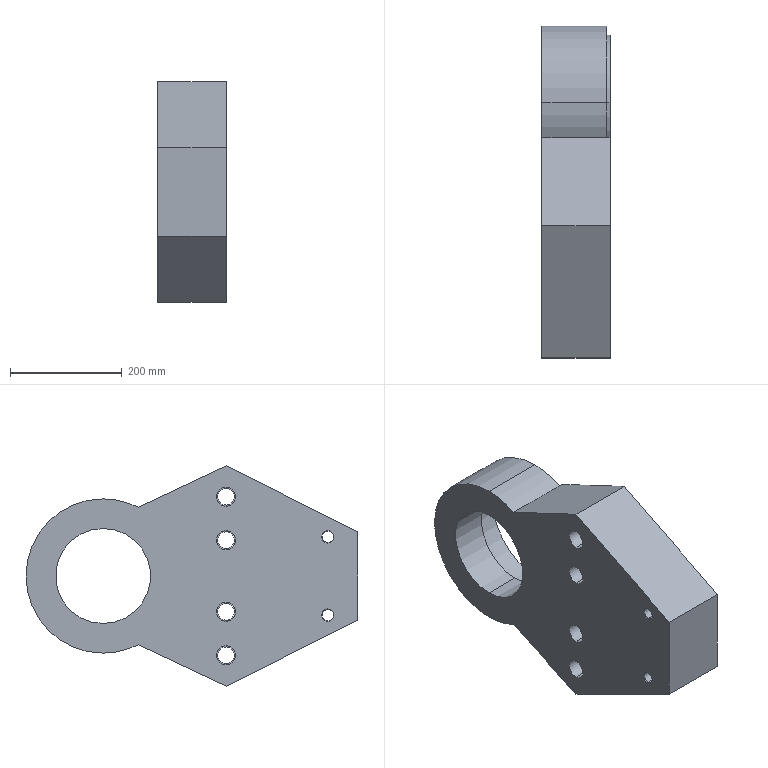Component | SolidWorks | Bracket-1 | 1 solid | 51 faces | box 122 x 594 x 395 mm | volume 15525976 mm3 | cylinder 32 | plane 15 | cone 4 | commonest cylinder face diameters 34 x8 30 x8 20 x4 276 x4 245 x2 221 x2 226 x2 170 x2
build123d program:
from build123d import *

# Parameters (mm, degrees)
BOSS_EXTRUDE1_DEPTH  = 122
SKETCH5_R            = 138
BOSS_EXTRUDE2_DEPTH  = 122
SKETCH2_R            = 85
CUT_EXTRUDE1_2_DEPTH = 512.69
SKETCH3_R            = 113
CUT_EXTRUDE2_DEPTH   = 48.5
SKETCH4_R            = 110.5
CUT_EXTRUDE3_DEPTH   = 8
CUT_EXTRUDE4_START   = 6.4
SKETCH6_R            = 138
SKETCH6_R_2          = 122.5
CUT_EXTRUDE4_DEPTH   = 6.4
M30_TAPPED_HOLE1_D   = 30
M20_TAPPED_HOLE1_D   = 20
SKETCH1_R            = 17
CUT_EXTRUDE1_DEPTH   = 33
CHAMFER1_SIZE        = 1


with BuildPart() as part:
    # Sketch1_2 → Boss-Extrude1 (new body)
    with BuildSketch(Plane.XY):
        Polygon((-93.5, 0), (93.5, 0), (197.5, 220), (78.811, 456), (-78.811, 456), (-197.5, 220), align=None)
    extrude(amount=BOSS_EXTRUDE1_DEPTH)

    # Sketch5 → Boss-Extrude2 (add)
    with BuildSketch(Plane(origin=(0, 0, 0), x_dir=(-1, 0, 0), z_dir=(0, 0, -1))):
        Circle(SKETCH5_R)
    extrude(amount=-BOSS_EXTRUDE2_DEPTH)

    # Sketch2 → Cut-Extrude1_2 (cut, through all)
    with BuildSketch(Plane(origin=(0, 0, 0), x_dir=(-1, 0, 0), z_dir=(0, 0, -1))):
        Circle(SKETCH2_R)
    extrude(amount=-CUT_EXTRUDE1_2_DEPTH, mode=Mode.SUBTRACT)

    # Sketch3 → Cut-Extrude2 (cut)
    with BuildSketch(Plane.XY.offset(122)):
        Circle(SKETCH3_R)
    extrude(amount=-CUT_EXTRUDE2_DEPTH, mode=Mode.SUBTRACT)

    # Sketch4 → Cut-Extrude3 (cut)
    with BuildSketch(Plane.XY.offset(73.5)):
        Circle(SKETCH4_R)
    extrude(amount=-CUT_EXTRUDE3_DEPTH, mode=Mode.SUBTRACT)

    # Sketch6 → Cut-Extrude4 (cut)
    with BuildSketch(Plane(origin=(0, 0, 122), x_dir=(-1, 0, 0), z_dir=(0, 0, -1)).offset(CUT_EXTRUDE4_START)):
        Circle(SKETCH6_R)
        Circle(SKETCH6_R_2, mode=Mode.SUBTRACT)
    extrude(amount=-CUT_EXTRUDE4_DEPTH, mode=Mode.SUBTRACT)

    # M30 Tapped Hole1 (through all)
    with Locations(Plane(origin=(0, 0, 0), x_dir=(-1, 0, 0), z_dir=(0, 0, -1))):
        with Locations((64, 220), (-64, 220), (-142, 220), (142, 220)):
            Hole(M30_TAPPED_HOLE1_D / 2)

    # M20 Tapped Hole1 (through all)
    with Locations(Plane(origin=(0, 0, 0), x_dir=(-1, 0, 0), z_dir=(0, 0, -1))):
        with Locations((70, 402), (-70, 402)):
            Hole(M20_TAPPED_HOLE1_D / 2)

    # Sketch1 → Cut-Extrude1 (cut)
    with BuildSketch(Plane(origin=(0, 0, 0), x_dir=(-1, 0, 0), z_dir=(0, 0, -1))):
        with Locations((-64, 220)):
            Circle(SKETCH1_R)
        with Locations((64, 220)):
            Circle(SKETCH1_R)
        with Locations((-142, 220)):
            Circle(SKETCH1_R)
        with Locations((142, 220)):
            Circle(SKETCH1_R)
    extrude(amount=-CUT_EXTRUDE1_DEPTH, mode=Mode.SUBTRACT)

    # Chamfer1
    chamfer1_edges = [part.edges().sort_by_distance(p)[0] for p in [
        (-80, 402, 0),
        (60, 402, 0),
    ]]
    chamfer(chamfer1_edges, length=CHAMFER1_SIZE)


solid = part.part

# Placed as in the assembly
solid = solid.moved(Location((-199.5, 0, 0), (180, 90, 0)))